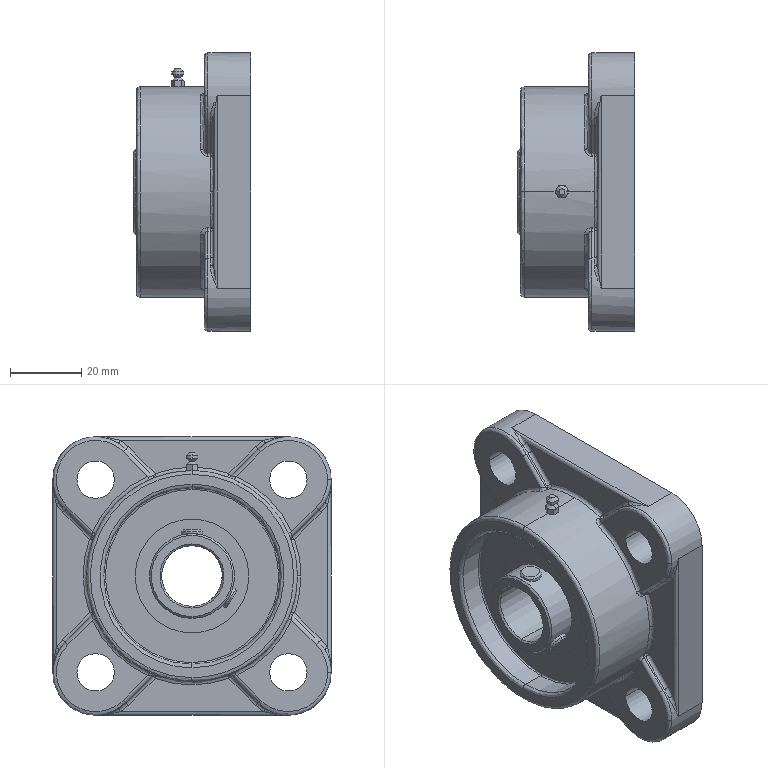Component | SolidWorks | SquarePillowBlockBearingUCFU203-3 | 1 solid | 196 faces | volume 87804 mm3 | cylinder 70 | spline 59 | plane 39 | cone 28 | commonest cylinder face diameters 2 x30 10.5 x8 6 x8 24 x6 49.5 x4 31.9 x4 23.8 x4 59 x2